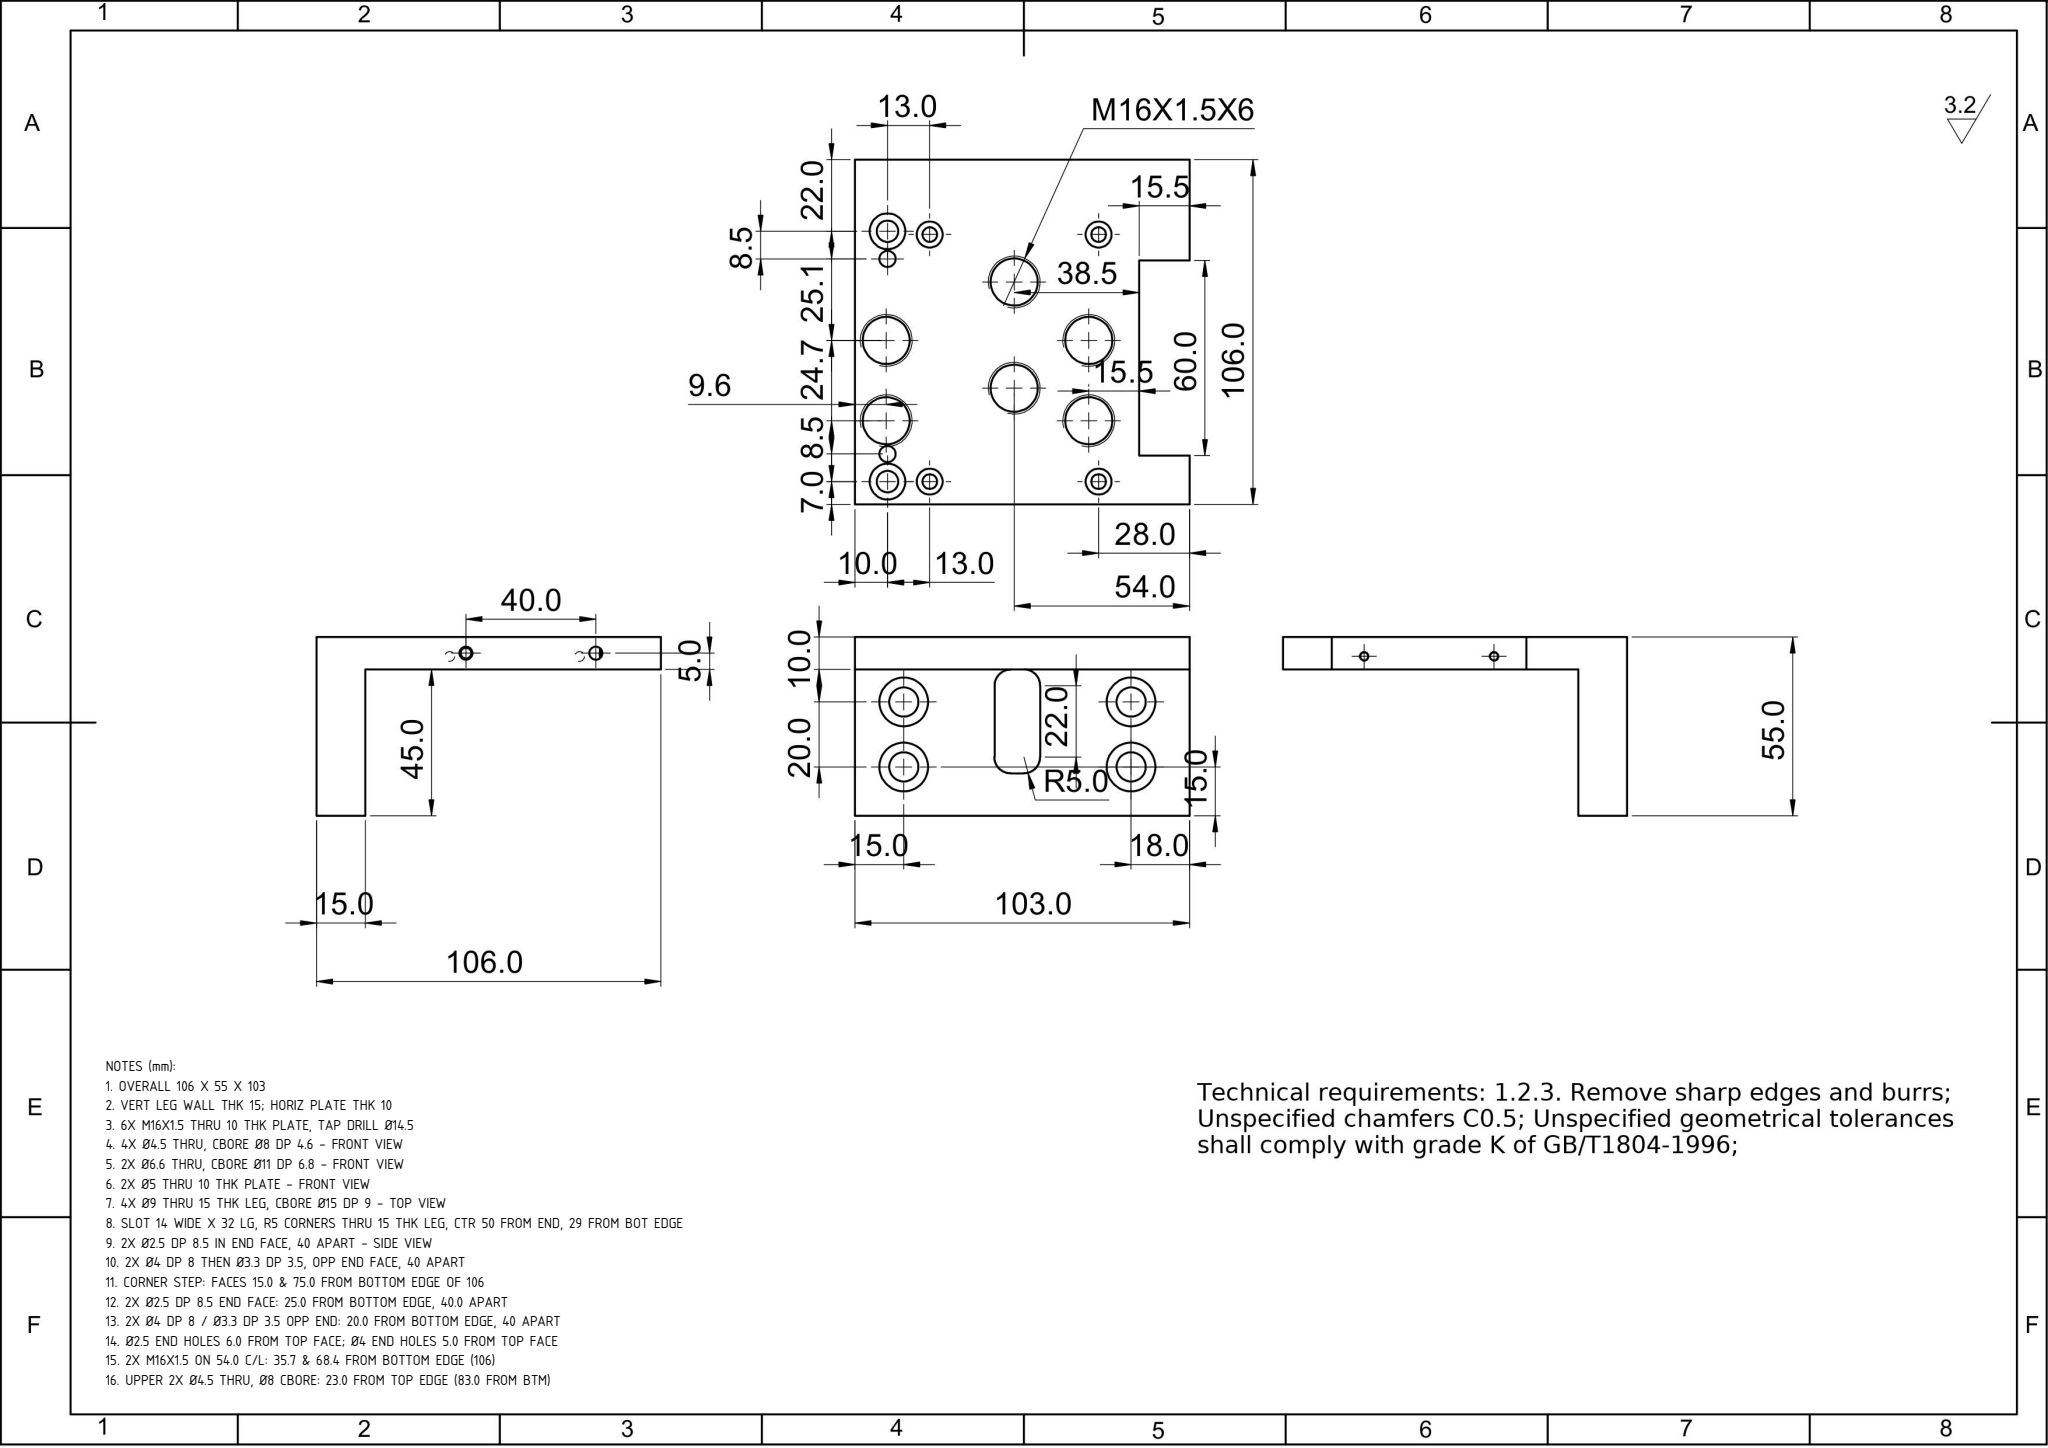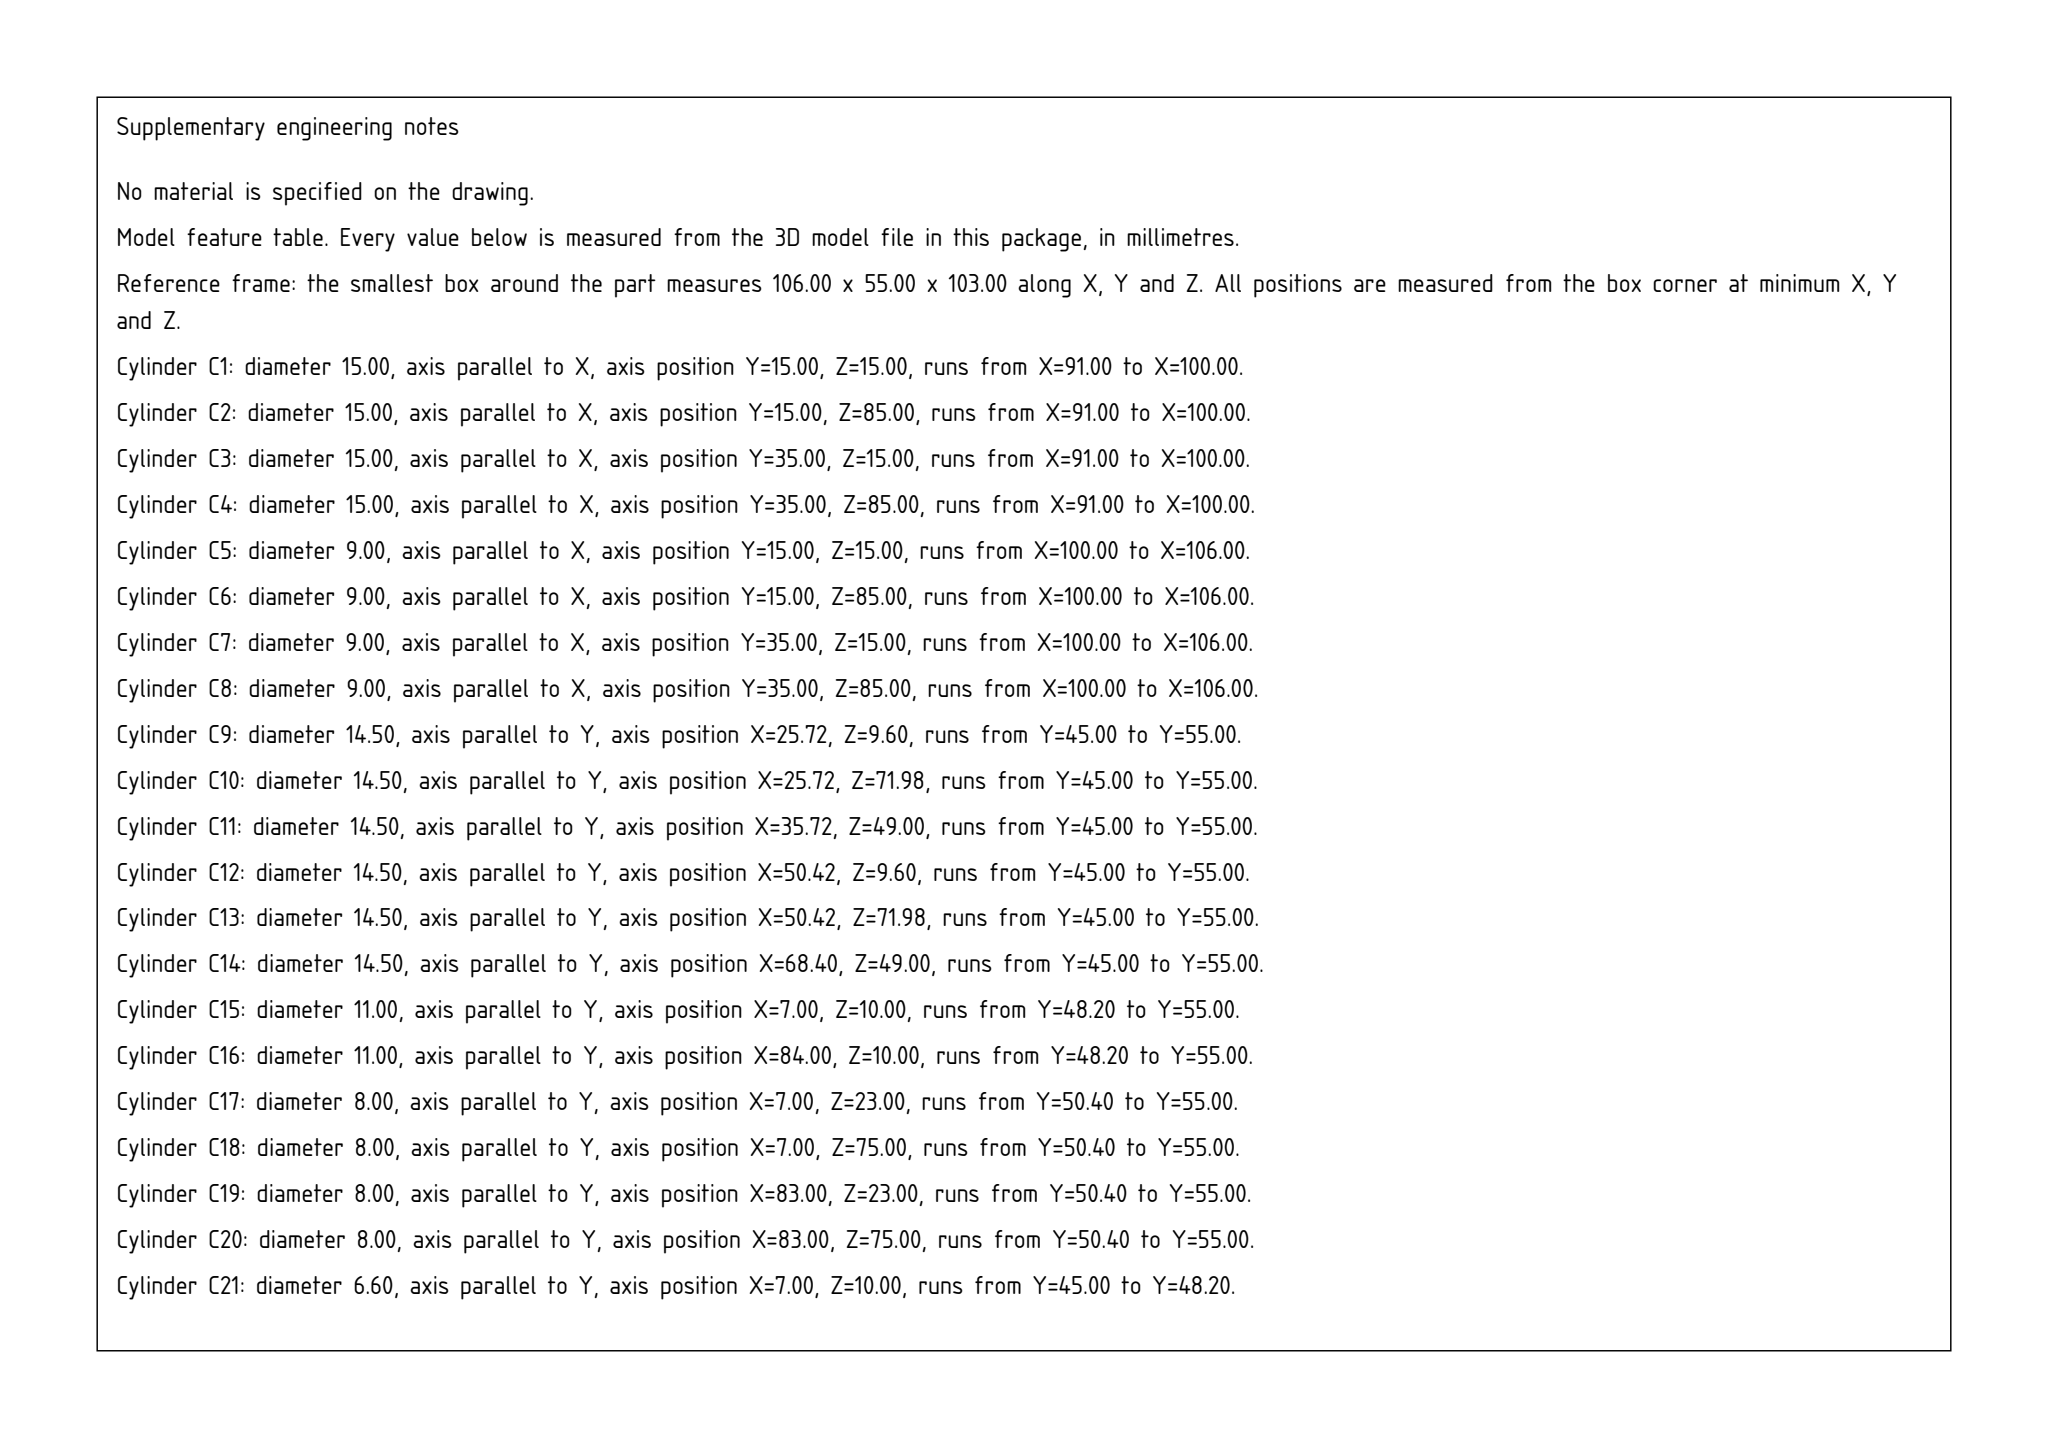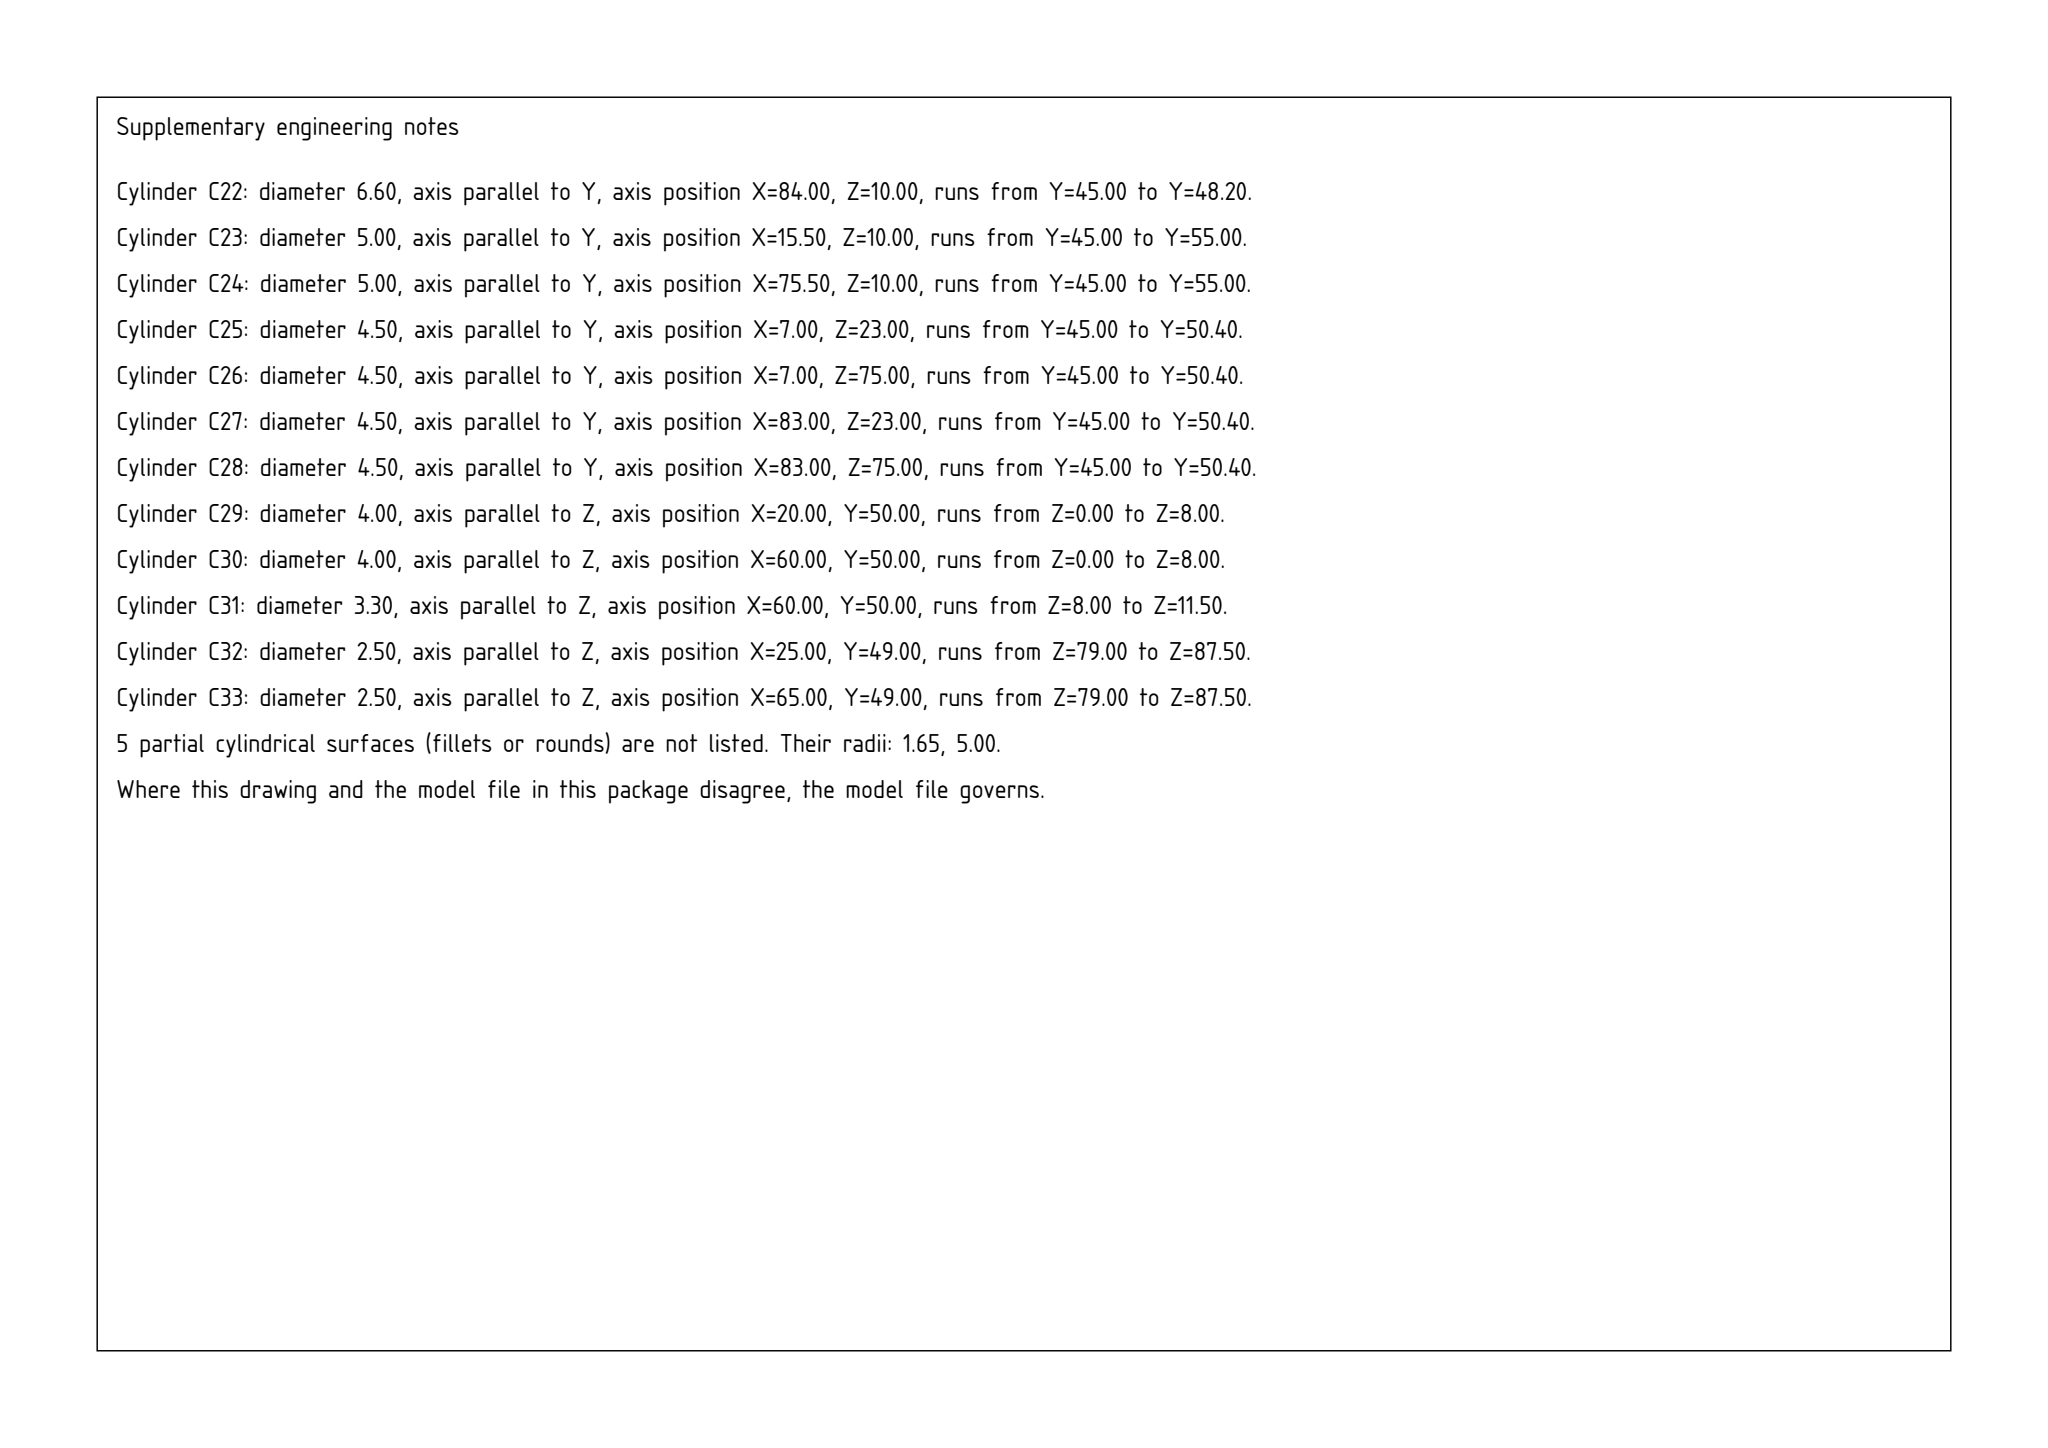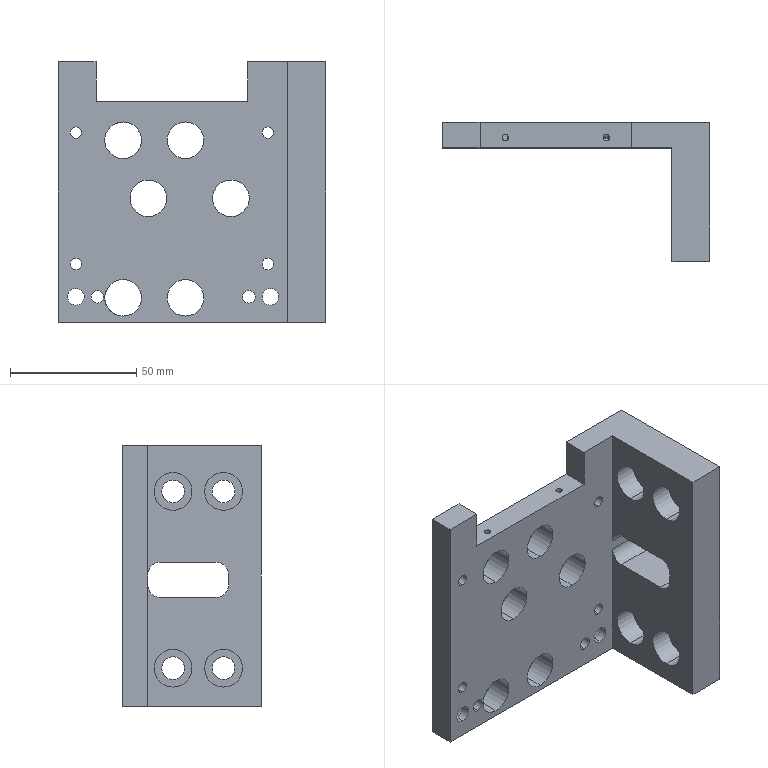Part | SolidWorks | mm | 1 solid | 105 faces | box 106 x 55 x 103 mm | volume 141752 mm3 | cylinder 71 | plane 27 | cone 7 | commonest cylinder face diameters 14.5 x12 15 x8 9 x8 8 x8 4.5 x8 5 x4 4 x4 2.5 x4
Drawing notes:
OVERALL 106 X 55 X 103 | from the solid: bbox_xyz [106.0, 55.0, 103.0]
VERT LEG WALL THK 15; HORIZ PLATE THK 10 | from the solid: x planes 0 and 15 (leg); y planes 45 and 55 (plate) in 106x55x103 bbox
6X M16X1.5 THRU 10 THK PLATE, TAP DRILL Ø14.5 | from the solid: 6 cyl dia 14.5 axis y L=10 at (25.72,9.6),(25.72,71.98),(35.72,49),(50.42,9.6),(50.42,71.98),(68.4,49); plate y=45..55
4X Ø4.5 THRU, CBORE Ø8 DP 4.6 - FRONT VIEW | from the solid: dia 4.5 axis y L=5.4 + dia 8.0 axis y L=4.6 at (x,z)=(7,23),(7,75),(83,23),(83,75); 5.4+4.6=10 thk
2X Ø6.6 THRU, CBORE Ø11 DP 6.8 - FRONT VIEW | from the solid: dia 6.6 axis y L=3.2 + dia 11.0 axis y L=6.8 at (x,z)=(7,10),(84,10); 3.2+6.8=10 thk
2X Ø5 THRU 10 THK PLATE - FRONT VIEW | from the solid: dia 5.0 axis y L=10 at (x,z)=(15.5,10),(75.5,10)
4X Ø9 THRU 15 THK LEG, CBORE Ø15 DP 9 - TOP VIEW | from the solid: dia 9.0 axis x L=6 + dia 15.0 axis x L=9 at (y,z)=(15,15),(15,85),(35,15),(35,85); leg x=0..15
SLOT 14 WIDE X 32 LG, R5 CORNERS THRU 15 THK LEG, CTR 50 FROM END, 29 FROM BOT EDGE | from the solid: four dia 10 axis x L=15 at (y,z)=(18,48),(18,52),(40,48),(40,52); planes y13/y45 -> ctr 29, z43/z57 -> ctr 50
2X Ø2.5 DP 8.5 IN END FACE, 40 APART - SIDE VIEW | from the solid: dia 2.5 axis z L=8.5 at (x,y)=(25,49),(65,49); 118 deg drill point
2X Ø4 DP 8 THEN Ø3.3 DP 3.5, OPP END FACE, 40 APART | from the solid: dia 4.0 axis z L=8 and dia 3.3 axis z L=3.5 at (x,y)=(20,50),(60,50); 118 deg point
CORNER STEP: FACES 15.0 & 75.0 FROM BOTTOM EDGE OF 106 | from the solid: axis_planes x=15.0 and x=75.0 (60.0 apart = 60.0 notch height), bbox x=106
2X Ø2.5 DP 8.5 END FACE: 25.0 FROM BOTTOM EDGE, 40.0 APART | from the solid: cyl Ø2.5 axis z at x=25.0 and x=65.0, len 8.5
2X Ø4 DP 8 / Ø3.3 DP 3.5 OPP END: 20.0 FROM BOTTOM EDGE, 40 APART | from the solid: cyl Ø4 len 8 and Ø3.3 len 3.5 axis z at x=20.0 and x=60.0
Ø2.5 END HOLES 6.0 FROM TOP FACE; Ø4 END HOLES 5.0 FROM TOP FACE | from the solid: Ø2.5 at y=49.0, Ø4/Ø3.3 at y=50.0, bbox y=55.0
2X M16X1.5 ON 54.0 C/L: 35.7 & 68.4 FROM BOTTOM EDGE (106) | from the solid: cyl Ø14.5 axis y at x=35.72 z=49.0 and x=68.4 z=49.0
UPPER 2X Ø4.5 THRU, Ø8 CBORE: 23.0 FROM TOP EDGE (83.0 FROM BTM) | from the solid: Ø4.5 y-axis holes at x=83.0 (z=23.0 & 75.0); Ø8 CBORE same axes; bbox x=106 so 106-83=23.0 from top edge; Ø6.6/Ø11 row at x=84.0 = 22.0 from top